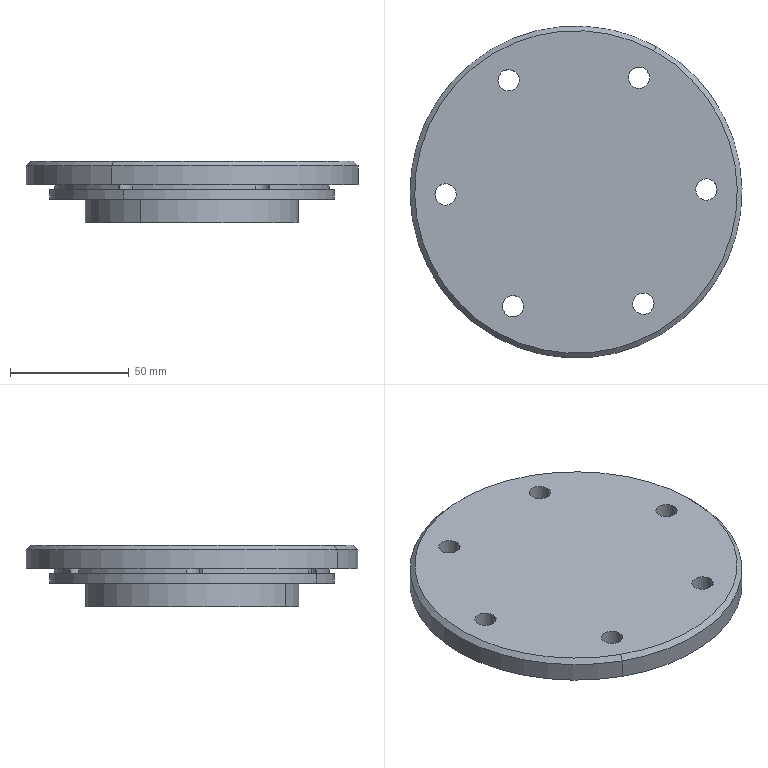Component | SolidWorks | OutputAxisEndCover2-0717-1 | 1 solid | 34 faces | volume 224229 mm3 | cylinder 26 | plane 6 | cone 2 | commonest cylinder face diameters 9 x12 116 x6 82 x2 90 x2 140 x2 120 x2